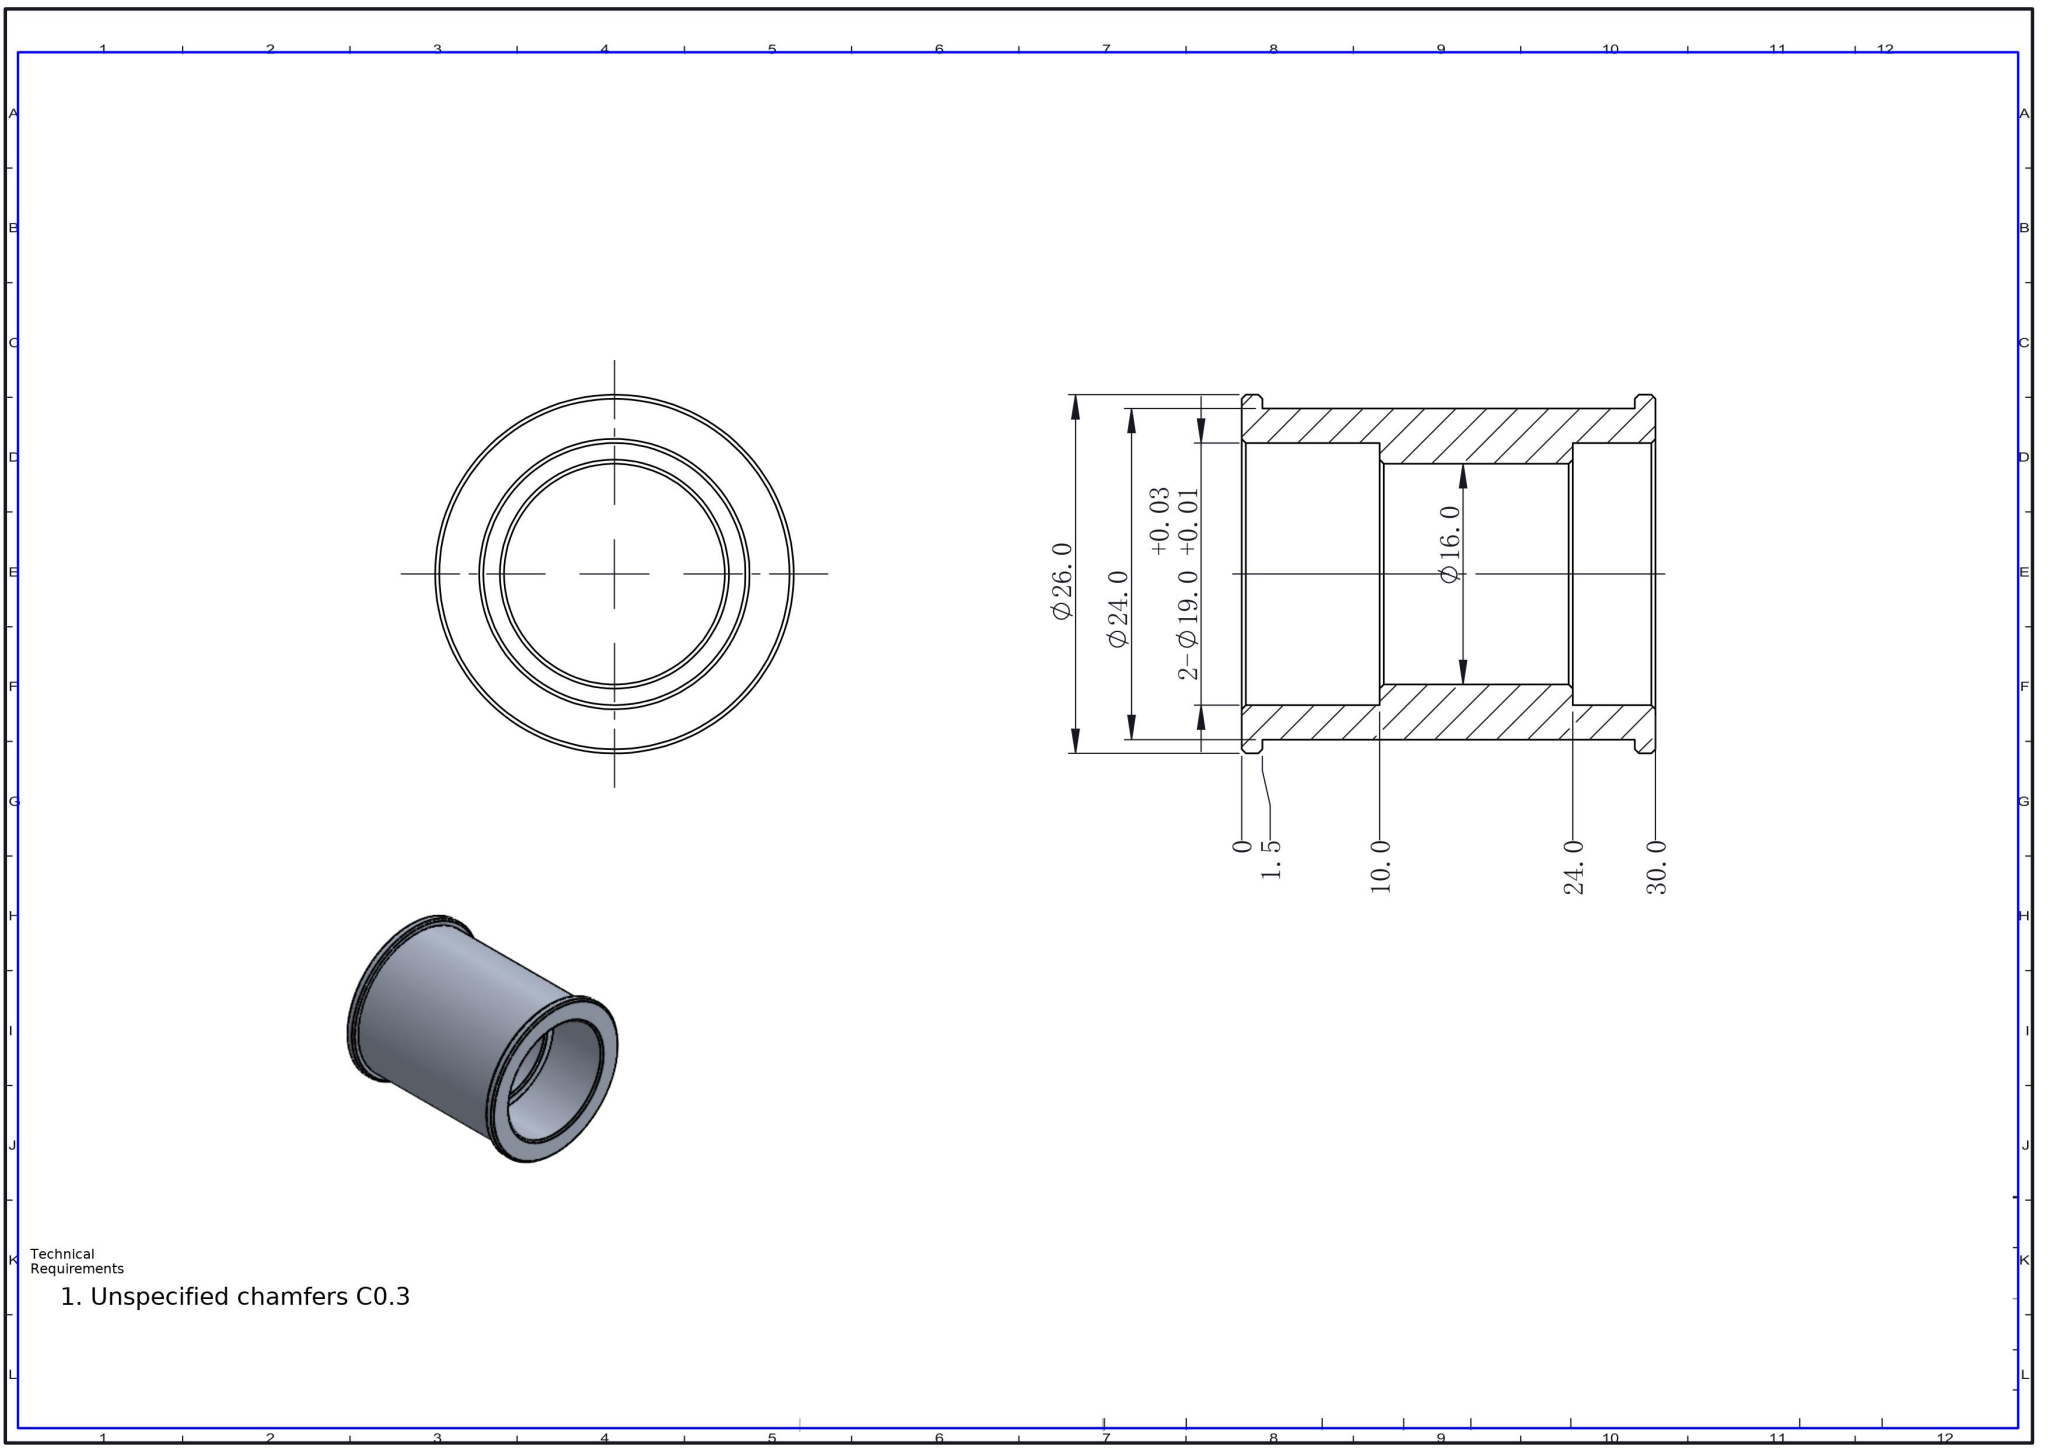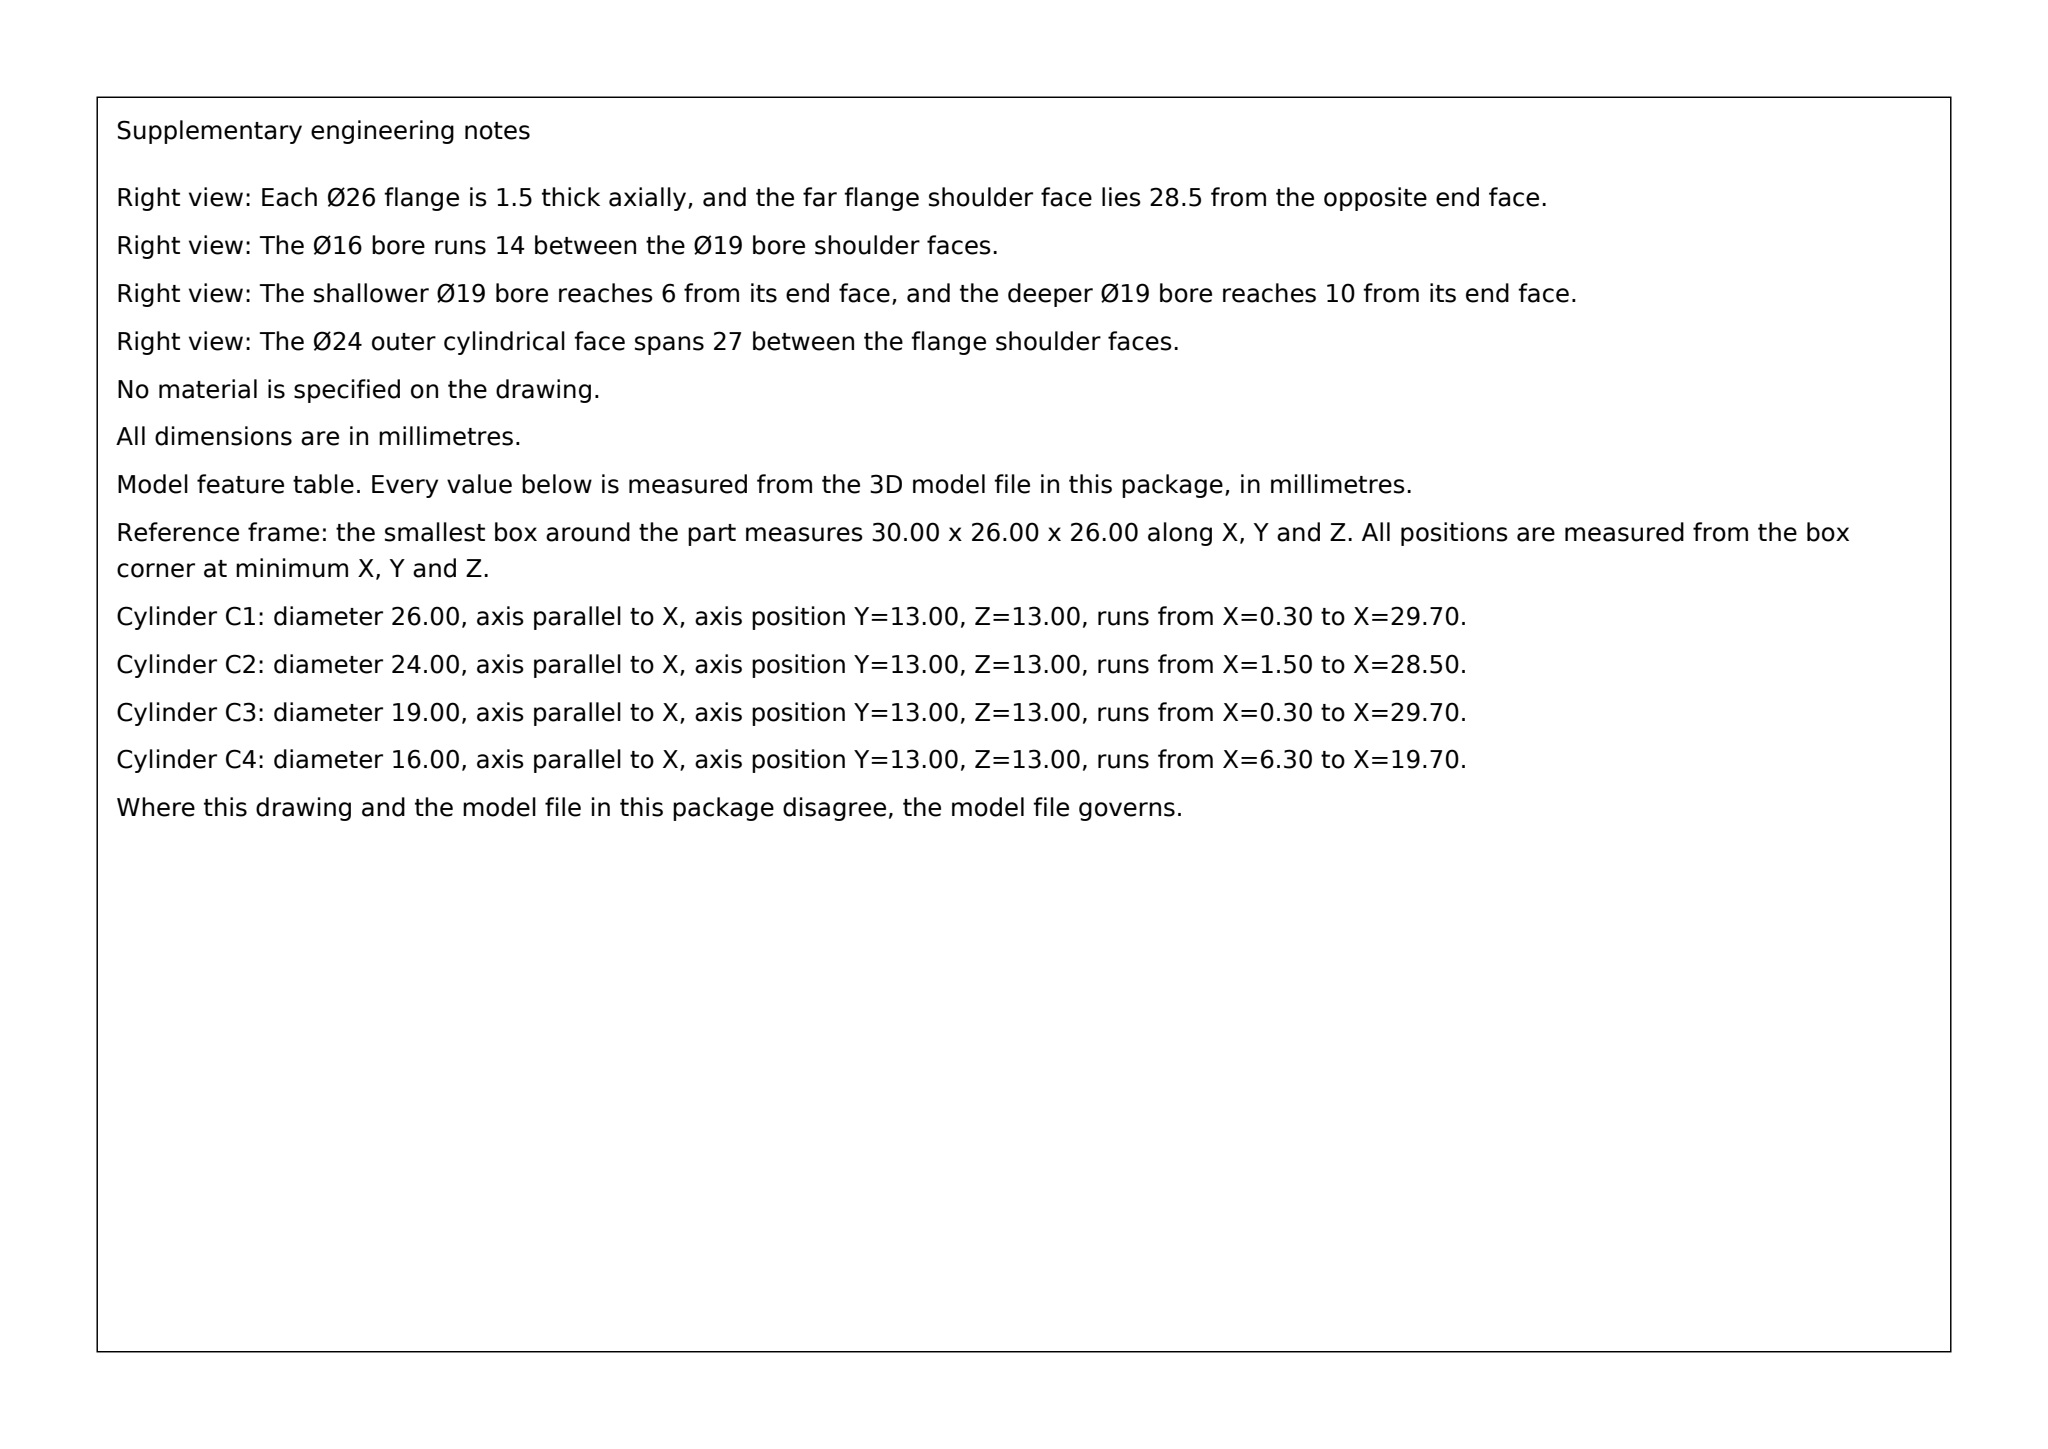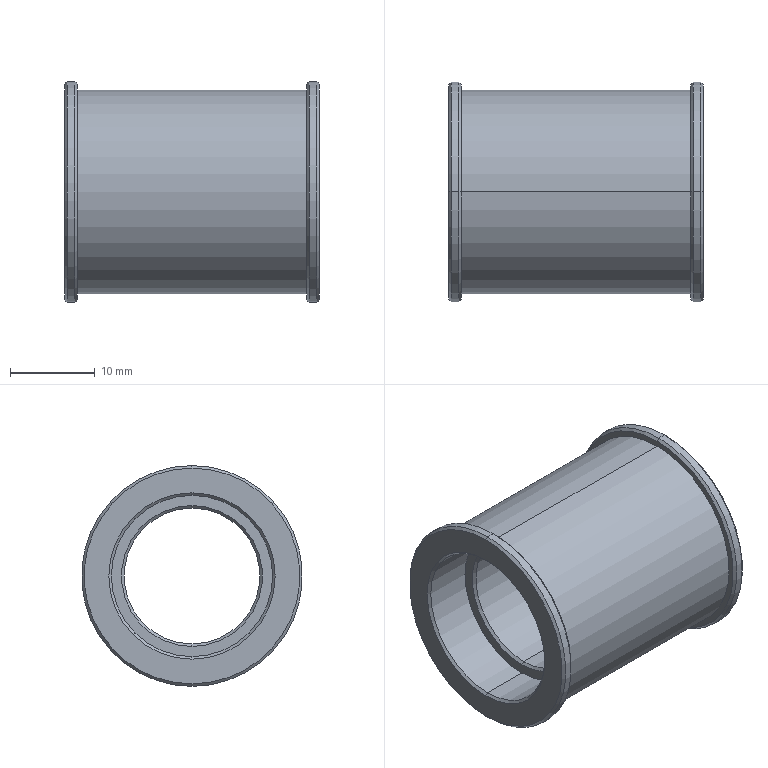Part | SolidWorks | mm | 1 solid | 34 faces | box 30 x 26 x 26 mm | volume 6431 mm3 | cone 16 | cylinder 12 | plane 6 | commonest cylinder face diameters 19 x4 26 x4 24 x2 16 x2
Drawing notes:
Ø26 COLLAR 1.5 WIDE EA END (0-1.5 & 28.5-30), C0.3 CHAM | from the solid: Ø26 cyl on x-axis at both ends; planes x=0/1.5 and x=28.5/30; 90 deg cones ref dia 26 & 25.4 (4 ea) give C0.3 breaks; Ø24 body 27 long between
build123d program:
from build123d import *

# Parameters (mm, degrees)
CHAMFER1_SIZE = 0.3


with BuildPart() as part:
    # Sketch1 → Revolve1 (revolve)
    with BuildSketch(Plane.XY, mode=Mode.PRIVATE) as revolve1_sk:
        Polygon((7, 8), (-7, 8), (-7, 9.5), (-13, 9.5), (-13, 13), (-11.5, 13), (-11.5, 12), (15.5, 12), (15.5, 13), (17, 13), (17, 9.5), (7, 9.5), align=None)
    revolve(revolve1_sk.sketch.rotate(Axis((0, 0, 0), (1, 0, 0)), 90), axis=Axis((0, 0, 0), (1, 0, 0)))

    # Chamfer1
    chamfer1_edges = [part.edges().sort_by_distance(p)[0] for p in [
        (17, 0, -13),
        (15.5, 0, -13),
        (-11.5, 0, -13),
        (-13, 0, -13),
        (-13, 0, -9.5),
        (-7, 0, -8),
        (7, 0, -8),
        (17, 0, -9.5),
    ]]
    chamfer(chamfer1_edges, length=CHAMFER1_SIZE)


solid = part.part
STEP:
#1=CARTESIAN_POINT('',(-13.,0.,12.7));
#2=VERTEX_POINT('',#1);
#3=CARTESIAN_POINT('',(-13.,0.,-12.7));
#4=VERTEX_POINT('',#3);
#5=CARTESIAN_POINT('',(-13.,0.,0.));
#6=DIRECTION('',(-1.,0.,0.));
#7=DIRECTION('',(0.,0.,-1.));
#8=AXIS2_PLACEMENT_3D('',#5,#6,#7);
#9=CIRCLE('',#8,12.7);
#10=EDGE_CURVE('',#2,#4,#9,.T.);
#11=ORIENTED_EDGE('',*,*,#10,.F.);
#12=CARTESIAN_POINT('',(-12.7,0.,13.));
#13=VERTEX_POINT('',#12);
#14=CARTESIAN_POINT('',(-13.,0.,12.7));
#15=DIRECTION('',(0.7071,0.,0.7071));
#16=VECTOR('',#15,1000.);
#17=LINE('',#14,#16);
#18=EDGE_CURVE('',#2,#13,#17,.T.);
#19=ORIENTED_EDGE('',*,*,#18,.T.);
#20=CARTESIAN_POINT('',(-12.7,0.,-13.));
#21=VERTEX_POINT('',#20);
#22=CARTESIAN_POINT('',(-12.7,0.,0.));
#23=DIRECTION('',(1.,0.,0.));
#24=DIRECTION('',(0.,0.,-1.));
#25=AXIS2_PLACEMENT_3D('',#22,#23,#24);
#26=CIRCLE('',#25,13.);
#27=EDGE_CURVE('',#21,#13,#26,.T.);
#28=ORIENTED_EDGE('',*,*,#27,.F.);
#29=CARTESIAN_POINT('',(-13.,0.,-12.7));
#30=DIRECTION('',(0.7071,0.,-0.7071));
#31=VECTOR('',#30,1000.);
#32=LINE('',#29,#31);
#33=EDGE_CURVE('',#4,#21,#32,.T.);
#34=ORIENTED_EDGE('',*,*,#33,.F.);
#35=EDGE_LOOP('',(#11,#19,#28,#34));
#36=FACE_OUTER_BOUND('',#35,.T.);
#37=CARTESIAN_POINT('',(-13.,0.,0.));
#38=DIRECTION('',(1.,0.,0.));
#39=DIRECTION('',(0.,0.,-1.));
#40=AXIS2_PLACEMENT_3D('',#37,#38,#39);
#41=CONICAL_SURFACE('',#40,12.7,0.7854);
#42=ADVANCED_FACE('',(#36),#41,.T.);
#43=CARTESIAN_POINT('',(-12.7,0.,-9.5));
#44=VERTEX_POINT('',#43);
#45=CARTESIAN_POINT('',(-12.7,0.,9.5));
#46=VERTEX_POINT('',#45);
#47=CARTESIAN_POINT('',(-12.7,0.,0.));
#48=DIRECTION('',(-1.,0.,0.));
#49=DIRECTION('',(0.,0.,-1.));
#50=AXIS2_PLACEMENT_3D('',#47,#48,#49);
#51=CIRCLE('',#50,9.5);
#52=EDGE_CURVE('',#44,#46,#51,.T.);
#53=ORIENTED_EDGE('',*,*,#52,.F.);
#54=CARTESIAN_POINT('',(-13.,0.,-9.8));
#55=VERTEX_POINT('',#54);
#56=CARTESIAN_POINT('',(-12.7,0.,-9.5));
#57=DIRECTION('',(-0.7071,0.,-0.7071));
#58=VECTOR('',#57,1000.);
#59=LINE('',#56,#58);
#60=EDGE_CURVE('',#44,#55,#59,.T.);
#61=ORIENTED_EDGE('',*,*,#60,.T.);
#62=CARTESIAN_POINT('',(-13.,0.,9.8));
#63=VERTEX_POINT('',#62);
#64=CARTESIAN_POINT('',(-13.,0.,0.));
#65=DIRECTION('',(1.,0.,0.));
#66=DIRECTION('',(0.,0.,-1.));
#67=AXIS2_PLACEMENT_3D('',#64,#65,#66);
#68=CIRCLE('',#67,9.8);
#69=EDGE_CURVE('',#63,#55,#68,.T.);
#70=ORIENTED_EDGE('',*,*,#69,.F.);
#71=CARTESIAN_POINT('',(-12.7,0.,9.5));
#72=DIRECTION('',(-0.7071,0.,0.7071));
#73=VECTOR('',#72,1000.);
#74=LINE('',#71,#73);
#75=EDGE_CURVE('',#46,#63,#74,.T.);
#76=ORIENTED_EDGE('',*,*,#75,.F.);
#77=EDGE_LOOP('',(#53,#61,#70,#76));
#78=FACE_OUTER_BOUND('',#77,.T.);
#79=CARTESIAN_POINT('',(-12.7,0.,0.));
#80=DIRECTION('',(-1.,0.,0.));
#81=DIRECTION('',(0.,0.,1.));
#82=AXIS2_PLACEMENT_3D('',#79,#80,#81);
#83=CONICAL_SURFACE('',#82,9.5,0.7854);
#84=ADVANCED_FACE('',(#78),#83,.F.);
#85=CARTESIAN_POINT('',(-6.7,0.,-8.));
#86=VERTEX_POINT('',#85);
#87=CARTESIAN_POINT('',(-6.7,0.,8.));
#88=VERTEX_POINT('',#87);
#89=CARTESIAN_POINT('',(-6.7,0.,0.));
#90=DIRECTION('',(-1.,0.,0.));
#91=DIRECTION('',(0.,0.,-1.));
#92=AXIS2_PLACEMENT_3D('',#89,#90,#91);
#93=CIRCLE('',#92,8.);
#94=EDGE_CURVE('',#86,#88,#93,.T.);
#95=ORIENTED_EDGE('',*,*,#94,.F.);
#96=CARTESIAN_POINT('',(-7.,0.,-8.3));
#97=VERTEX_POINT('',#96);
#98=CARTESIAN_POINT('',(-6.7,0.,-8.));
#99=DIRECTION('',(-0.7071,0.,-0.7071));
#100=VECTOR('',#99,1000.);
#101=LINE('',#98,#100);
#102=EDGE_CURVE('',#86,#97,#101,.T.);
#103=ORIENTED_EDGE('',*,*,#102,.T.);
#104=CARTESIAN_POINT('',(-7.,0.,8.3));
#105=VERTEX_POINT('',#104);
#106=CARTESIAN_POINT('',(-7.,0.,0.));
#107=DIRECTION('',(1.,0.,0.));
#108=DIRECTION('',(0.,0.,-1.));
#109=AXIS2_PLACEMENT_3D('',#106,#107,#108);
#110=CIRCLE('',#109,8.3);
#111=EDGE_CURVE('',#105,#97,#110,.T.);
#112=ORIENTED_EDGE('',*,*,#111,.F.);
#113=CARTESIAN_POINT('',(-6.7,0.,8.));
#114=DIRECTION('',(-0.7071,0.,0.7071));
#115=VECTOR('',#114,1000.);
#116=LINE('',#113,#115);
#117=EDGE_CURVE('',#88,#105,#116,.T.);
#118=ORIENTED_EDGE('',*,*,#117,.F.);
#119=EDGE_LOOP('',(#95,#103,#112,#118));
#120=FACE_OUTER_BOUND('',#119,.T.);
#121=CARTESIAN_POINT('',(-6.7,0.,0.));
#122=DIRECTION('',(-1.,0.,0.));
#123=DIRECTION('',(0.,0.,1.));
#124=AXIS2_PLACEMENT_3D('',#121,#122,#123);
#125=CONICAL_SURFACE('',#124,8.,0.7854);
#126=ADVANCED_FACE('',(#120),#125,.F.);
#127=CARTESIAN_POINT('',(16.7,0.,9.5));
#128=VERTEX_POINT('',#127);
#129=CARTESIAN_POINT('',(16.7,0.,-9.5));
#130=VERTEX_POINT('',#129);
#131=CARTESIAN_POINT('',(16.7,0.,0.));
#132=DIRECTION('',(1.,0.,0.));
#133=DIRECTION('',(0.,0.,1.));
#134=AXIS2_PLACEMENT_3D('',#131,#132,#133);
#135=CIRCLE('',#134,9.5);
#136=EDGE_CURVE('',#128,#130,#135,.T.);
#137=ORIENTED_EDGE('',*,*,#136,.F.);
#138=CARTESIAN_POINT('',(17.,0.,9.8));
#139=VERTEX_POINT('',#138);
#140=CARTESIAN_POINT('',(17.,0.,9.8));
#141=DIRECTION('',(0.7071,0.,0.7071));
#142=VECTOR('',#141,1000.);
#143=LINE('',#140,#142);
#144=EDGE_CURVE('',#128,#139,#143,.T.);
#145=ORIENTED_EDGE('',*,*,#144,.T.);
#146=CARTESIAN_POINT('',(17.,0.,-9.8));
#147=VERTEX_POINT('',#146);
#148=CARTESIAN_POINT('',(17.,0.,0.));
#149=DIRECTION('',(-1.,0.,0.));
#150=DIRECTION('',(0.,0.,1.));
#151=AXIS2_PLACEMENT_3D('',#148,#149,#150);
#152=CIRCLE('',#151,9.8);
#153=EDGE_CURVE('',#147,#139,#152,.T.);
#154=ORIENTED_EDGE('',*,*,#153,.F.);
#155=CARTESIAN_POINT('',(17.,0.,-9.8));
#156=DIRECTION('',(0.7071,0.,-0.7071));
#157=VECTOR('',#156,1000.);
#158=LINE('',#155,#157);
#159=EDGE_CURVE('',#130,#147,#158,.T.);
#160=ORIENTED_EDGE('',*,*,#159,.F.);
#161=EDGE_LOOP('',(#137,#145,#154,#160));
#162=FACE_OUTER_BOUND('',#161,.T.);
#163=CARTESIAN_POINT('',(17.,0.,0.));
#164=DIRECTION('',(1.,0.,0.));
#165=DIRECTION('',(0.,0.,-1.));
#166=AXIS2_PLACEMENT_3D('',#163,#164,#165);
#167=CONICAL_SURFACE('',#166,9.8,0.7854);
#168=ADVANCED_FACE('',(#162),#167,.F.);
#169=CARTESIAN_POINT('',(17.,0.,-12.7));
#170=VERTEX_POINT('',#169);
#171=CARTESIAN_POINT('',(17.,0.,12.7));
#172=VERTEX_POINT('',#171);
#173=CARTESIAN_POINT('',(17.,0.,0.));
#174=DIRECTION('',(1.,0.,0.));
#175=DIRECTION('',(0.,0.,1.));
#176=AXIS2_PLACEMENT_3D('',#173,#174,#175);
#177=CIRCLE('',#176,12.7);
#178=EDGE_CURVE('',#170,#172,#177,.T.);
#179=ORIENTED_EDGE('',*,*,#178,.F.);
#180=CARTESIAN_POINT('',(16.7,0.,-13.));
#181=VERTEX_POINT('',#180);
#182=CARTESIAN_POINT('',(16.7,0.,-13.));
#183=DIRECTION('',(-0.7071,0.,-0.7071));
#184=VECTOR('',#183,1000.);
#185=LINE('',#182,#184);
#186=EDGE_CURVE('',#170,#181,#185,.T.);
#187=ORIENTED_EDGE('',*,*,#186,.T.);
#188=CARTESIAN_POINT('',(16.7,0.,13.));
#189=VERTEX_POINT('',#188);
#190=CARTESIAN_POINT('',(16.7,0.,0.));
#191=DIRECTION('',(-1.,0.,0.));
#192=DIRECTION('',(0.,0.,1.));
#193=AXIS2_PLACEMENT_3D('',#190,#191,#192);
#194=CIRCLE('',#193,13.);
#195=EDGE_CURVE('',#189,#181,#194,.T.);
#196=ORIENTED_EDGE('',*,*,#195,.F.);
#197=CARTESIAN_POINT('',(16.7,0.,13.));
#198=DIRECTION('',(-0.7071,0.,0.7071));
#199=VECTOR('',#198,1000.);
#200=LINE('',#197,#199);
#201=EDGE_CURVE('',#172,#189,#200,.T.);
#202=ORIENTED_EDGE('',*,*,#201,.F.);
#203=EDGE_LOOP('',(#179,#187,#196,#202));
#204=FACE_OUTER_BOUND('',#203,.T.);
#205=CARTESIAN_POINT('',(16.7,0.,0.));
#206=DIRECTION('',(-1.,0.,0.));
#207=DIRECTION('',(0.,0.,1.));
#208=AXIS2_PLACEMENT_3D('',#205,#206,#207);
#209=CONICAL_SURFACE('',#208,13.,0.7854);
#210=ADVANCED_FACE('',(#204),#209,.T.);
#211=CARTESIAN_POINT('',(15.5,0.,12.7));
#212=VERTEX_POINT('',#211);
#213=CARTESIAN_POINT('',(15.5,0.,-12.7));
#214=VERTEX_POINT('',#213);
#215=CARTESIAN_POINT('',(15.5,0.,0.));
#216=DIRECTION('',(-1.,0.,0.));
#217=DIRECTION('',(0.,0.,-1.));
#218=AXIS2_PLACEMENT_3D('',#215,#216,#217);
#219=CIRCLE('',#218,12.7);
#220=EDGE_CURVE('',#212,#214,#219,.T.);
#221=ORIENTED_EDGE('',*,*,#220,.F.);
#222=CARTESIAN_POINT('',(15.8,0.,13.));
#223=VERTEX_POINT('',#222);
#224=CARTESIAN_POINT('',(15.5,0.,12.7));
#225=DIRECTION('',(0.7071,0.,0.7071));
#226=VECTOR('',#225,1000.);
#227=LINE('',#224,#226);
#228=EDGE_CURVE('',#212,#223,#227,.T.);
#229=ORIENTED_EDGE('',*,*,#228,.T.);
#230=CARTESIAN_POINT('',(15.8,0.,-13.));
#231=VERTEX_POINT('',#230);
#232=CARTESIAN_POINT('',(15.8,0.,0.));
#233=DIRECTION('',(1.,0.,0.));
#234=DIRECTION('',(0.,0.,-1.));
#235=AXIS2_PLACEMENT_3D('',#232,#233,#234);
#236=CIRCLE('',#235,13.);
#237=EDGE_CURVE('',#231,#223,#236,.T.);
#238=ORIENTED_EDGE('',*,*,#237,.F.);
#239=CARTESIAN_POINT('',(15.5,0.,-12.7));
#240=DIRECTION('',(0.7071,0.,-0.7071));
#241=VECTOR('',#240,1000.);
#242=LINE('',#239,#241);
#243=EDGE_CURVE('',#214,#231,#242,.T.);
#244=ORIENTED_EDGE('',*,*,#243,.F.);
#245=EDGE_LOOP('',(#221,#229,#238,#244));
#246=FACE_OUTER_BOUND('',#245,.T.);
#247=CARTESIAN_POINT('',(15.5,0.,0.));
#248=DIRECTION('',(1.,0.,0.));
#249=DIRECTION('',(0.,0.,-1.));
#250=AXIS2_PLACEMENT_3D('',#247,#248,#249);
#251=CONICAL_SURFACE('',#250,12.7,0.7854);
#252=ADVANCED_FACE('',(#246),#251,.T.);
#253=CARTESIAN_POINT('',(6.7,0.,8.));
#254=VERTEX_POINT('',#253);
#255=CARTESIAN_POINT('',(6.7,0.,-8.));
#256=VERTEX_POINT('',#255);
#257=CARTESIAN_POINT('',(6.7,0.,0.));
#258=DIRECTION('',(1.,0.,0.));
#259=DIRECTION('',(0.,0.,1.));
#260=AXIS2_PLACEMENT_3D('',#257,#258,#259);
#261=CIRCLE('',#260,8.);
#262=EDGE_CURVE('',#254,#256,#261,.T.);
#263=ORIENTED_EDGE('',*,*,#262,.F.);
#264=CARTESIAN_POINT('',(7.,0.,8.3));
#265=VERTEX_POINT('',#264);
#266=CARTESIAN_POINT('',(7.,0.,8.3));
#267=DIRECTION('',(0.7071,0.,0.7071));
#268=VECTOR('',#267,1000.);
#269=LINE('',#266,#268);
#270=EDGE_CURVE('',#254,#265,#269,.T.);
#271=ORIENTED_EDGE('',*,*,#270,.T.);
#272=CARTESIAN_POINT('',(7.,0.,-8.3));
#273=VERTEX_POINT('',#272);
#274=CARTESIAN_POINT('',(7.,0.,0.));
#275=DIRECTION('',(-1.,0.,0.));
#276=DIRECTION('',(0.,0.,1.));
#277=AXIS2_PLACEMENT_3D('',#274,#275,#276);
#278=CIRCLE('',#277,8.3);
#279=EDGE_CURVE('',#273,#265,#278,.T.);
#280=ORIENTED_EDGE('',*,*,#279,.F.);
#281=CARTESIAN_POINT('',(7.,0.,-8.3));
#282=DIRECTION('',(0.7071,0.,-0.7071));
#283=VECTOR('',#282,1000.);
#284=LINE('',#281,#283);
#285=EDGE_CURVE('',#256,#273,#284,.T.);
#286=ORIENTED_EDGE('',*,*,#285,.F.);
#287=EDGE_LOOP('',(#263,#271,#280,#286));
#288=FACE_OUTER_BOUND('',#287,.T.);
#289=CARTESIAN_POINT('',(7.,0.,0.));
#290=DIRECTION('',(1.,0.,0.));
#291=DIRECTION('',(0.,0.,-1.));
#292=AXIS2_PLACEMENT_3D('',#289,#290,#291);
#293=CONICAL_SURFACE('',#292,8.3,0.7854);
#294=ADVANCED_FACE('',(#288),#293,.F.);
#295=CARTESIAN_POINT('',(-11.5,0.,-12.7));
#296=VERTEX_POINT('',#295);
#297=CARTESIAN_POINT('',(-11.5,0.,12.7));
#298=VERTEX_POINT('',#297);
#299=CARTESIAN_POINT('',(-11.5,0.,0.));
#300=DIRECTION('',(1.,0.,0.));
#301=DIRECTION('',(0.,0.,1.));
#302=AXIS2_PLACEMENT_3D('',#299,#300,#301);
#303=CIRCLE('',#302,12.7);
#304=EDGE_CURVE('',#296,#298,#303,.T.);
#305=ORIENTED_EDGE('',*,*,#304,.F.);
#306=CARTESIAN_POINT('',(-11.8,0.,-13.));
#307=VERTEX_POINT('',#306);
#308=CARTESIAN_POINT('',(-11.8,0.,-13.));
#309=DIRECTION('',(-0.7071,0.,-0.7071));
#310=VECTOR('',#309,1000.);
#311=LINE('',#308,#310);
#312=EDGE_CURVE('',#296,#307,#311,.T.);
#313=ORIENTED_EDGE('',*,*,#312,.T.);
#314=CARTESIAN_POINT('',(-11.8,0.,13.));
#315=VERTEX_POINT('',#314);
#316=CARTESIAN_POINT('',(-11.8,0.,0.));
#317=DIRECTION('',(-1.,0.,0.));
#318=DIRECTION('',(0.,0.,1.));
#319=AXIS2_PLACEMENT_3D('',#316,#317,#318);
#320=CIRCLE('',#319,13.);
#321=EDGE_CURVE('',#315,#307,#320,.T.);
#322=ORIENTED_EDGE('',*,*,#321,.F.);
#323=CARTESIAN_POINT('',(-11.8,0.,13.));
#324=DIRECTION('',(-0.7071,0.,0.7071));
#325=VECTOR('',#324,1000.);
#326=LINE('',#323,#325);
#327=EDGE_CURVE('',#298,#315,#326,.T.);
#328=ORIENTED_EDGE('',*,*,#327,.F.);
#329=EDGE_LOOP('',(#305,#313,#322,#328));
#330=FACE_OUTER_BOUND('',#329,.T.);
#331=CARTESIAN_POINT('',(-11.8,0.,0.));
#332=DIRECTION('',(-1.,0.,0.));
#333=DIRECTION('',(0.,0.,1.));
#334=AXIS2_PLACEMENT_3D('',#331,#332,#333);
#335=CONICAL_SURFACE('',#334,13.,0.7854);
#336=ADVANCED_FACE('',(#330),#335,.T.);
#337=ORIENTED_EDGE('',*,*,#136,.T.);
#338=CARTESIAN_POINT('',(7.,0.,-9.5));
#339=VERTEX_POINT('',#338);
#340=CARTESIAN_POINT('',(0.,0.,-9.5));
#341=DIRECTION('',(-1.,0.,0.));
#342=VECTOR('',#341,1000.);
#343=LINE('',#340,#342);
#344=EDGE_CURVE('',#130,#339,#343,.T.);
#345=ORIENTED_EDGE('',*,*,#344,.T.);
#346=CARTESIAN_POINT('',(7.,0.,9.5));
#347=VERTEX_POINT('',#346);
#348=CARTESIAN_POINT('',(7.,0.,0.));
#349=DIRECTION('',(-1.,0.,0.));
#350=DIRECTION('',(0.,0.,1.));
#351=AXIS2_PLACEMENT_3D('',#348,#349,#350);
#352=CIRCLE('',#351,9.5);
#353=EDGE_CURVE('',#339,#347,#352,.T.);
#354=ORIENTED_EDGE('',*,*,#353,.T.);
#355=CARTESIAN_POINT('',(0.,0.,9.5));
#356=DIRECTION('',(-1.,0.,0.));
#357=VECTOR('',#356,1000.);
#358=LINE('',#355,#357);
#359=EDGE_CURVE('',#128,#347,#358,.T.);
#360=ORIENTED_EDGE('',*,*,#359,.F.);
#361=EDGE_LOOP('',(#337,#345,#354,#360));
#362=FACE_OUTER_BOUND('',#361,.T.);
#363=CARTESIAN_POINT('',(0.,0.,0.));
#364=DIRECTION('',(-1.,0.,0.));
#365=DIRECTION('',(0.,0.,1.));
#366=AXIS2_PLACEMENT_3D('',#363,#364,#365);
#367=CYLINDRICAL_SURFACE('',#366,9.5);
#368=ADVANCED_FACE('',(#362),#367,.F.);
#369=ORIENTED_EDGE('',*,*,#195,.T.);
#370=CARTESIAN_POINT('',(0.,0.,-13.));
#371=DIRECTION('',(-1.,0.,0.));
#372=VECTOR('',#371,1000.);
#373=LINE('',#370,#372);
#374=EDGE_CURVE('',#181,#231,#373,.T.);
#375=ORIENTED_EDGE('',*,*,#374,.T.);
#376=ORIENTED_EDGE('',*,*,#237,.T.);
#377=CARTESIAN_POINT('',(0.,0.,13.));
#378=DIRECTION('',(-1.,0.,0.));
#379=VECTOR('',#378,1000.);
#380=LINE('',#377,#379);
#381=EDGE_CURVE('',#189,#223,#380,.T.);
#382=ORIENTED_EDGE('',*,*,#381,.F.);
#383=EDGE_LOOP('',(#369,#375,#376,#382));
#384=FACE_OUTER_BOUND('',#383,.T.);
#385=CARTESIAN_POINT('',(0.,0.,0.));
#386=DIRECTION('',(-1.,0.,0.));
#387=DIRECTION('',(0.,0.,1.));
#388=AXIS2_PLACEMENT_3D('',#385,#386,#387);
#389=CYLINDRICAL_SURFACE('',#388,13.);
#390=ADVANCED_FACE('',(#384),#389,.T.);
#391=CARTESIAN_POINT('',(15.5,0.,12.));
#392=VERTEX_POINT('',#391);
#393=CARTESIAN_POINT('',(15.5,0.,-12.));
#394=VERTEX_POINT('',#393);
#395=CARTESIAN_POINT('',(15.5,0.,0.));
#396=DIRECTION('',(-1.,0.,0.));
#397=DIRECTION('',(0.,0.,1.));
#398=AXIS2_PLACEMENT_3D('',#395,#396,#397);
#399=CIRCLE('',#398,12.);
#400=EDGE_CURVE('',#392,#394,#399,.T.);
#401=ORIENTED_EDGE('',*,*,#400,.T.);
#402=CARTESIAN_POINT('',(-11.5,0.,-12.));
#403=VERTEX_POINT('',#402);
#404=CARTESIAN_POINT('',(0.,0.,-12.));
#405=DIRECTION('',(-1.,0.,0.));
#406=VECTOR('',#405,1000.);
#407=LINE('',#404,#406);
#408=EDGE_CURVE('',#394,#403,#407,.T.);
#409=ORIENTED_EDGE('',*,*,#408,.T.);
#410=CARTESIAN_POINT('',(-11.5,0.,12.));
#411=VERTEX_POINT('',#410);
#412=CARTESIAN_POINT('',(-11.5,0.,0.));
#413=DIRECTION('',(-1.,0.,0.));
#414=DIRECTION('',(0.,0.,1.));
#415=AXIS2_PLACEMENT_3D('',#412,#413,#414);
#416=CIRCLE('',#415,12.);
#417=EDGE_CURVE('',#411,#403,#416,.T.);
#418=ORIENTED_EDGE('',*,*,#417,.F.);
#419=CARTESIAN_POINT('',(0.,0.,12.));
#420=DIRECTION('',(-1.,0.,0.));
#421=VECTOR('',#420,1000.);
#422=LINE('',#419,#421);
#423=EDGE_CURVE('',#392,#411,#422,.T.);
#424=ORIENTED_EDGE('',*,*,#423,.F.);
#425=EDGE_LOOP('',(#401,#409,#418,#424));
#426=FACE_OUTER_BOUND('',#425,.T.);
#427=CARTESIAN_POINT('',(0.,0.,0.));
#428=DIRECTION('',(-1.,0.,0.));
#429=DIRECTION('',(0.,0.,1.));
#430=AXIS2_PLACEMENT_3D('',#427,#428,#429);
#431=CYLINDRICAL_SURFACE('',#430,12.);
#432=ADVANCED_FACE('',(#426),#431,.T.);
#433=ORIENTED_EDGE('',*,*,#321,.T.);
#434=CARTESIAN_POINT('',(0.,0.,-13.));
#435=DIRECTION('',(-1.,0.,0.));
#436=VECTOR('',#435,1000.);
#437=LINE('',#434,#436);
#438=EDGE_CURVE('',#307,#21,#437,.T.);
#439=ORIENTED_EDGE('',*,*,#438,.T.);
#440=ORIENTED_EDGE('',*,*,#27,.T.);
#441=CARTESIAN_POINT('',(0.,0.,13.));
#442=DIRECTION('',(-1.,0.,0.));
#443=VECTOR('',#442,1000.);
#444=LINE('',#441,#443);
#445=EDGE_CURVE('',#315,#13,#444,.T.);
#446=ORIENTED_EDGE('',*,*,#445,.F.);
#447=EDGE_LOOP('',(#433,#439,#440,#446));
#448=FACE_OUTER_BOUND('',#447,.T.);
#449=CARTESIAN_POINT('',(0.,0.,0.));
#450=DIRECTION('',(-1.,0.,0.));
#451=DIRECTION('',(0.,0.,1.));
#452=AXIS2_PLACEMENT_3D('',#449,#450,#451);
#453=CYLINDRICAL_SURFACE('',#452,13.);
#454=ADVANCED_FACE('',(#448),#453,.T.);
#455=CARTESIAN_POINT('',(-7.,0.,-9.5));
#456=VERTEX_POINT('',#455);
#457=CARTESIAN_POINT('',(-7.,0.,9.5));
#458=VERTEX_POINT('',#457);
#459=CARTESIAN_POINT('',(-7.,0.,0.));
#460=DIRECTION('',(-1.,0.,0.));
#461=DIRECTION('',(0.,0.,1.));
#462=AXIS2_PLACEMENT_3D('',#459,#460,#461);
#463=CIRCLE('',#462,9.5);
#464=EDGE_CURVE('',#456,#458,#463,.T.);
#465=ORIENTED_EDGE('',*,*,#464,.F.);
#466=CARTESIAN_POINT('',(0.,0.,-9.5));
#467=DIRECTION('',(-1.,0.,0.));
#468=VECTOR('',#467,1000.);
#469=LINE('',#466,#468);
#470=EDGE_CURVE('',#456,#44,#469,.T.);
#471=ORIENTED_EDGE('',*,*,#470,.T.);
#472=ORIENTED_EDGE('',*,*,#52,.T.);
#473=CARTESIAN_POINT('',(0.,0.,9.5));
#474=DIRECTION('',(-1.,0.,0.));
#475=VECTOR('',#474,1000.);
#476=LINE('',#473,#475);
#477=EDGE_CURVE('',#458,#46,#476,.T.);
#478=ORIENTED_EDGE('',*,*,#477,.F.);
#479=EDGE_LOOP('',(#465,#471,#472,#478));
#480=FACE_OUTER_BOUND('',#479,.T.);
#481=CARTESIAN_POINT('',(0.,0.,0.));
#482=DIRECTION('',(-1.,0.,0.));
#483=DIRECTION('',(0.,0.,1.));
#484=AXIS2_PLACEMENT_3D('',#481,#482,#483);
#485=CYLINDRICAL_SURFACE('',#484,9.5);
#486=ADVANCED_FACE('',(#480),#485,.F.);
#487=ORIENTED_EDGE('',*,*,#262,.T.);
#488=CARTESIAN_POINT('',(0.,0.,-8.));
#489=DIRECTION('',(-1.,0.,0.));
#490=VECTOR('',#489,1000.);
#491=LINE('',#488,#490);
#492=EDGE_CURVE('',#256,#86,#491,.T.);
#493=ORIENTED_EDGE('',*,*,#492,.T.);
#494=ORIENTED_EDGE('',*,*,#94,.T.);
#495=CARTESIAN_POINT('',(0.,0.,8.));
#496=DIRECTION('',(-1.,0.,0.));
#497=VECTOR('',#496,1000.);
#498=LINE('',#495,#497);
#499=EDGE_CURVE('',#254,#88,#498,.T.);
#500=ORIENTED_EDGE('',*,*,#499,.F.);
#501=EDGE_LOOP('',(#487,#493,#494,#500));
#502=FACE_OUTER_BOUND('',#501,.T.);
#503=CARTESIAN_POINT('',(0.,0.,0.));
#504=DIRECTION('',(-1.,0.,0.));
#505=DIRECTION('',(0.,0.,1.));
#506=AXIS2_PLACEMENT_3D('',#503,#504,#505);
#507=CYLINDRICAL_SURFACE('',#506,8.);
#508=ADVANCED_FACE('',(#502),#507,.F.);
#509=ORIENTED_EDGE('',*,*,#279,.T.);
#510=CARTESIAN_POINT('',(7.,0.,0.));
#511=DIRECTION('',(-1.,0.,0.));
#512=DIRECTION('',(0.,0.,1.));
#513=AXIS2_PLACEMENT_3D('',#510,#511,#512);
#514=CIRCLE('',#513,8.3);
#515=EDGE_CURVE('',#265,#273,#514,.T.);
#516=ORIENTED_EDGE('',*,*,#515,.T.);
#517=EDGE_LOOP('',(#509,#516));
#518=FACE_BOUND('',#517,.T.);
#519=CARTESIAN_POINT('',(7.,0.,0.));
#520=DIRECTION('',(-1.,0.,0.));
#521=DIRECTION('',(0.,0.,1.));
#522=AXIS2_PLACEMENT_3D('',#519,#520,#521);
#523=CIRCLE('',#522,9.5);
#524=EDGE_CURVE('',#347,#339,#523,.T.);
#525=ORIENTED_EDGE('',*,*,#524,.F.);
#526=ORIENTED_EDGE('',*,*,#353,.F.);
#527=EDGE_LOOP('',(#525,#526));
#528=FACE_OUTER_BOUND('',#527,.T.);
#529=CARTESIAN_POINT('',(7.,9.5,0.));
#530=DIRECTION('',(-1.,0.,0.));
#531=DIRECTION('',(0.,0.,1.));
#532=AXIS2_PLACEMENT_3D('',#529,#530,#531);
#533=PLANE('',#532);
#534=ADVANCED_FACE('',(#518,#528),#533,.F.);
#535=ORIENTED_EDGE('',*,*,#492,.F.);
#536=CARTESIAN_POINT('',(6.7,0.,0.));
#537=DIRECTION('',(1.,0.,0.));
#538=DIRECTION('',(0.,0.,1.));
#539=AXIS2_PLACEMENT_3D('',#536,#537,#538);
#540=CIRCLE('',#539,8.);
#541=EDGE_CURVE('',#256,#254,#540,.T.);
#542=ORIENTED_EDGE('',*,*,#541,.T.);
#543=ORIENTED_EDGE('',*,*,#499,.T.);
#544=CARTESIAN_POINT('',(-6.7,0.,0.));
#545=DIRECTION('',(-1.,0.,0.));
#546=DIRECTION('',(0.,0.,-1.));
#547=AXIS2_PLACEMENT_3D('',#544,#545,#546);
#548=CIRCLE('',#547,8.);
#549=EDGE_CURVE('',#88,#86,#548,.T.);
#550=ORIENTED_EDGE('',*,*,#549,.T.);
#551=EDGE_LOOP('',(#535,#542,#543,#550));
#552=FACE_OUTER_BOUND('',#551,.T.);
#553=CARTESIAN_POINT('',(0.,0.,0.));
#554=DIRECTION('',(-1.,0.,0.));
#555=DIRECTION('',(0.,0.,1.));
#556=AXIS2_PLACEMENT_3D('',#553,#554,#555);
#557=CYLINDRICAL_SURFACE('',#556,8.);
#558=ADVANCED_FACE('',(#552),#557,.F.);
#559=ORIENTED_EDGE('',*,*,#111,.T.);
#560=CARTESIAN_POINT('',(-7.,0.,0.));
#561=DIRECTION('',(1.,0.,0.));
#562=DIRECTION('',(0.,0.,-1.));
#563=AXIS2_PLACEMENT_3D('',#560,#561,#562);
#564=CIRCLE('',#563,8.3);
#565=EDGE_CURVE('',#97,#105,#564,.T.);
#566=ORIENTED_EDGE('',*,*,#565,.T.);
#567=EDGE_LOOP('',(#559,#566));
#568=FACE_BOUND('',#567,.T.);
#569=CARTESIAN_POINT('',(-7.,0.,0.));
#570=DIRECTION('',(-1.,0.,0.));
#571=DIRECTION('',(0.,0.,1.));
#572=AXIS2_PLACEMENT_3D('',#569,#570,#571);
#573=CIRCLE('',#572,9.5);
#574=EDGE_CURVE('',#458,#456,#573,.T.);
#575=ORIENTED_EDGE('',*,*,#574,.T.);
#576=ORIENTED_EDGE('',*,*,#464,.T.);
#577=EDGE_LOOP('',(#575,#576));
#578=FACE_OUTER_BOUND('',#577,.T.);
#579=CARTESIAN_POINT('',(-7.,8.,0.));
#580=DIRECTION('',(1.,0.,0.));
#581=DIRECTION('',(0.,0.,-1.));
#582=AXIS2_PLACEMENT_3D('',#579,#580,#581);
#583=PLANE('',#582);
#584=ADVANCED_FACE('',(#568,#578),#583,.F.);
#585=ORIENTED_EDGE('',*,*,#470,.F.);
#586=ORIENTED_EDGE('',*,*,#574,.F.);
#587=ORIENTED_EDGE('',*,*,#477,.T.);
#588=CARTESIAN_POINT('',(-12.7,0.,0.));
#589=DIRECTION('',(-1.,0.,0.));
#590=DIRECTION('',(0.,0.,-1.));
#591=AXIS2_PLACEMENT_3D('',#588,#589,#590);
#592=CIRCLE('',#591,9.5);
#593=EDGE_CURVE('',#46,#44,#592,.T.);
#594=ORIENTED_EDGE('',*,*,#593,.T.);
#595=EDGE_LOOP('',(#585,#586,#587,#594));
#596=FACE_OUTER_BOUND('',#595,.T.);
#597=CARTESIAN_POINT('',(0.,0.,0.));
#598=DIRECTION('',(-1.,0.,0.));
#599=DIRECTION('',(0.,0.,1.));
#600=AXIS2_PLACEMENT_3D('',#597,#598,#599);
#601=CYLINDRICAL_SURFACE('',#600,9.5);
#602=ADVANCED_FACE('',(#596),#601,.F.);
#603=ORIENTED_EDGE('',*,*,#69,.T.);
#604=CARTESIAN_POINT('',(-13.,0.,0.));
#605=DIRECTION('',(1.,0.,0.));
#606=DIRECTION('',(0.,0.,-1.));
#607=AXIS2_PLACEMENT_3D('',#604,#605,#606);
#608=CIRCLE('',#607,9.8);
#609=EDGE_CURVE('',#55,#63,#608,.T.);
#610=ORIENTED_EDGE('',*,*,#609,.T.);
#611=EDGE_LOOP('',(#603,#610));
#612=FACE_BOUND('',#611,.T.);
#613=CARTESIAN_POINT('',(-13.,0.,0.));
#614=DIRECTION('',(-1.,0.,0.));
#615=DIRECTION('',(0.,0.,-1.));
#616=AXIS2_PLACEMENT_3D('',#613,#614,#615);
#617=CIRCLE('',#616,12.7);
#618=EDGE_CURVE('',#4,#2,#617,.T.);
#619=ORIENTED_EDGE('',*,*,#618,.T.);
#620=ORIENTED_EDGE('',*,*,#10,.T.);
#621=EDGE_LOOP('',(#619,#620));
#622=FACE_OUTER_BOUND('',#621,.T.);
#623=CARTESIAN_POINT('',(-13.,9.5,0.));
#624=DIRECTION('',(1.,0.,0.));
#625=DIRECTION('',(0.,0.,-1.));
#626=AXIS2_PLACEMENT_3D('',#623,#624,#625);
#627=PLANE('',#626);
#628=ADVANCED_FACE('',(#612,#622),#627,.F.);
#629=ORIENTED_EDGE('',*,*,#438,.F.);
#630=CARTESIAN_POINT('',(-11.8,0.,0.));
#631=DIRECTION('',(-1.,0.,0.));
#632=DIRECTION('',(0.,0.,1.));
#633=AXIS2_PLACEMENT_3D('',#630,#631,#632);
#634=CIRCLE('',#633,13.);
#635=EDGE_CURVE('',#307,#315,#634,.T.);
#636=ORIENTED_EDGE('',*,*,#635,.T.);
#637=ORIENTED_EDGE('',*,*,#445,.T.);
#638=CARTESIAN_POINT('',(-12.7,0.,0.));
#639=DIRECTION('',(1.,0.,0.));
#640=DIRECTION('',(0.,0.,-1.));
#641=AXIS2_PLACEMENT_3D('',#638,#639,#640);
#642=CIRCLE('',#641,13.);
#643=EDGE_CURVE('',#13,#21,#642,.T.);
#644=ORIENTED_EDGE('',*,*,#643,.T.);
#645=EDGE_LOOP('',(#629,#636,#637,#644));
#646=FACE_OUTER_BOUND('',#645,.T.);
#647=CARTESIAN_POINT('',(0.,0.,0.));
#648=DIRECTION('',(-1.,0.,0.));
#649=DIRECTION('',(0.,0.,1.));
#650=AXIS2_PLACEMENT_3D('',#647,#648,#649);
#651=CYLINDRICAL_SURFACE('',#650,13.);
#652=ADVANCED_FACE('',(#646),#651,.T.);
#653=CARTESIAN_POINT('',(-11.5,0.,0.));
#654=DIRECTION('',(1.,0.,0.));
#655=DIRECTION('',(0.,0.,1.));
#656=AXIS2_PLACEMENT_3D('',#653,#654,#655);
#657=CIRCLE('',#656,12.7);
#658=EDGE_CURVE('',#298,#296,#657,.T.);
#659=ORIENTED_EDGE('',*,*,#658,.T.);
#660=ORIENTED_EDGE('',*,*,#304,.T.);
#661=EDGE_LOOP('',(#659,#660));
#662=FACE_OUTER_BOUND('',#661,.T.);
#663=ORIENTED_EDGE('',*,*,#417,.T.);
#664=CARTESIAN_POINT('',(-11.5,0.,0.));
#665=DIRECTION('',(-1.,0.,0.));
#666=DIRECTION('',(0.,0.,1.));
#667=AXIS2_PLACEMENT_3D('',#664,#665,#666);
#668=CIRCLE('',#667,12.);
#669=EDGE_CURVE('',#403,#411,#668,.T.);
#670=ORIENTED_EDGE('',*,*,#669,.T.);
#671=EDGE_LOOP('',(#663,#670));
#672=FACE_BOUND('',#671,.T.);
#673=CARTESIAN_POINT('',(-11.5,13.,0.));
#674=DIRECTION('',(-1.,0.,0.));
#675=DIRECTION('',(0.,0.,1.));
#676=AXIS2_PLACEMENT_3D('',#673,#674,#675);
#677=PLANE('',#676);
#678=ADVANCED_FACE('',(#662,#672),#677,.F.);
#679=ORIENTED_EDGE('',*,*,#408,.F.);
#680=CARTESIAN_POINT('',(15.5,0.,0.));
#681=DIRECTION('',(-1.,0.,0.));
#682=DIRECTION('',(0.,0.,1.));
#683=AXIS2_PLACEMENT_3D('',#680,#681,#682);
#684=CIRCLE('',#683,12.);
#685=EDGE_CURVE('',#394,#392,#684,.T.);
#686=ORIENTED_EDGE('',*,*,#685,.T.);
#687=ORIENTED_EDGE('',*,*,#423,.T.);
#688=ORIENTED_EDGE('',*,*,#669,.F.);
#689=EDGE_LOOP('',(#679,#686,#687,#688));
#690=FACE_OUTER_BOUND('',#689,.T.);
#691=CARTESIAN_POINT('',(0.,0.,0.));
#692=DIRECTION('',(-1.,0.,0.));
#693=DIRECTION('',(0.,0.,1.));
#694=AXIS2_PLACEMENT_3D('',#691,#692,#693);
#695=CYLINDRICAL_SURFACE('',#694,12.);
#696=ADVANCED_FACE('',(#690),#695,.T.);
#697=CARTESIAN_POINT('',(15.5,0.,0.));
#698=DIRECTION('',(-1.,0.,0.));
#699=DIRECTION('',(0.,0.,-1.));
#700=AXIS2_PLACEMENT_3D('',#697,#698,#699);
#701=CIRCLE('',#700,12.7);
#702=EDGE_CURVE('',#214,#212,#701,.T.);
#703=ORIENTED_EDGE('',*,*,#702,.T.);
#704=ORIENTED_EDGE('',*,*,#220,.T.);
#705=EDGE_LOOP('',(#703,#704));
#706=FACE_OUTER_BOUND('',#705,.T.);
#707=ORIENTED_EDGE('',*,*,#400,.F.);
#708=ORIENTED_EDGE('',*,*,#685,.F.);
#709=EDGE_LOOP('',(#707,#708));
#710=FACE_BOUND('',#709,.T.);
#711=CARTESIAN_POINT('',(15.5,12.,0.));
#712=DIRECTION('',(1.,0.,0.));
#713=DIRECTION('',(0.,0.,-1.));
#714=AXIS2_PLACEMENT_3D('',#711,#712,#713);
#715=PLANE('',#714);
#716=ADVANCED_FACE('',(#706,#710),#715,.F.);
#717=ORIENTED_EDGE('',*,*,#374,.F.);
#718=CARTESIAN_POINT('',(16.7,0.,0.));
#719=DIRECTION('',(-1.,0.,0.));
#720=DIRECTION('',(0.,0.,1.));
#721=AXIS2_PLACEMENT_3D('',#718,#719,#720);
#722=CIRCLE('',#721,13.);
#723=EDGE_CURVE('',#181,#189,#722,.T.);
#724=ORIENTED_EDGE('',*,*,#723,.T.);
#725=ORIENTED_EDGE('',*,*,#381,.T.);
#726=CARTESIAN_POINT('',(15.8,0.,0.));
#727=DIRECTION('',(1.,0.,0.));
#728=DIRECTION('',(0.,0.,-1.));
#729=AXIS2_PLACEMENT_3D('',#726,#727,#728);
#730=CIRCLE('',#729,13.);
#731=EDGE_CURVE('',#223,#231,#730,.T.);
#732=ORIENTED_EDGE('',*,*,#731,.T.);
#733=EDGE_LOOP('',(#717,#724,#725,#732));
#734=FACE_OUTER_BOUND('',#733,.T.);
#735=CARTESIAN_POINT('',(0.,0.,0.));
#736=DIRECTION('',(-1.,0.,0.));
#737=DIRECTION('',(0.,0.,1.));
#738=AXIS2_PLACEMENT_3D('',#735,#736,#737);
#739=CYLINDRICAL_SURFACE('',#738,13.);
#740=ADVANCED_FACE('',(#734),#739,.T.);
#741=CARTESIAN_POINT('',(17.,0.,0.));
#742=DIRECTION('',(1.,0.,0.));
#743=DIRECTION('',(0.,0.,1.));
#744=AXIS2_PLACEMENT_3D('',#741,#742,#743);
#745=CIRCLE('',#744,12.7);
#746=EDGE_CURVE('',#172,#170,#745,.T.);
#747=ORIENTED_EDGE('',*,*,#746,.T.);
#748=ORIENTED_EDGE('',*,*,#178,.T.);
#749=EDGE_LOOP('',(#747,#748));
#750=FACE_OUTER_BOUND('',#749,.T.);
#751=ORIENTED_EDGE('',*,*,#153,.T.);
#752=CARTESIAN_POINT('',(17.,0.,0.));
#753=DIRECTION('',(-1.,0.,0.));
#754=DIRECTION('',(0.,0.,1.));
#755=AXIS2_PLACEMENT_3D('',#752,#753,#754);
#756=CIRCLE('',#755,9.8);
#757=EDGE_CURVE('',#139,#147,#756,.T.);
#758=ORIENTED_EDGE('',*,*,#757,.T.);
#759=EDGE_LOOP('',(#751,#758));
#760=FACE_BOUND('',#759,.T.);
#761=CARTESIAN_POINT('',(17.,13.,0.));
#762=DIRECTION('',(-1.,0.,0.));
#763=DIRECTION('',(0.,0.,1.));
#764=AXIS2_PLACEMENT_3D('',#761,#762,#763);
#765=PLANE('',#764);
#766=ADVANCED_FACE('',(#750,#760),#765,.F.);
#767=ORIENTED_EDGE('',*,*,#344,.F.);
#768=CARTESIAN_POINT('',(16.7,0.,0.));
#769=DIRECTION('',(1.,0.,0.));
#770=DIRECTION('',(0.,0.,1.));
#771=AXIS2_PLACEMENT_3D('',#768,#769,#770);
#772=CIRCLE('',#771,9.5);
#773=EDGE_CURVE('',#130,#128,#772,.T.);
#774=ORIENTED_EDGE('',*,*,#773,.T.);
#775=ORIENTED_EDGE('',*,*,#359,.T.);
#776=ORIENTED_EDGE('',*,*,#524,.T.);
#777=EDGE_LOOP('',(#767,#774,#775,#776));
#778=FACE_OUTER_BOUND('',#777,.T.);
#779=CARTESIAN_POINT('',(0.,0.,0.));
#780=DIRECTION('',(-1.,0.,0.));
#781=DIRECTION('',(0.,0.,1.));
#782=AXIS2_PLACEMENT_3D('',#779,#780,#781);
#783=CYLINDRICAL_SURFACE('',#782,9.5);
#784=ADVANCED_FACE('',(#778),#783,.F.);
#785=ORIENTED_EDGE('',*,*,#312,.F.);
#786=ORIENTED_EDGE('',*,*,#658,.F.);
#787=ORIENTED_EDGE('',*,*,#327,.T.);
#788=ORIENTED_EDGE('',*,*,#635,.F.);
#789=EDGE_LOOP('',(#785,#786,#787,#788));
#790=FACE_OUTER_BOUND('',#789,.T.);
#791=CARTESIAN_POINT('',(-11.8,0.,0.));
#792=DIRECTION('',(-1.,0.,0.));
#793=DIRECTION('',(0.,0.,1.));
#794=AXIS2_PLACEMENT_3D('',#791,#792,#793);
#795=CONICAL_SURFACE('',#794,13.,0.7854);
#796=ADVANCED_FACE('',(#790),#795,.T.);
#797=ORIENTED_EDGE('',*,*,#270,.F.);
#798=ORIENTED_EDGE('',*,*,#541,.F.);
#799=ORIENTED_EDGE('',*,*,#285,.T.);
#800=ORIENTED_EDGE('',*,*,#515,.F.);
#801=EDGE_LOOP('',(#797,#798,#799,#800));
#802=FACE_OUTER_BOUND('',#801,.T.);
#803=CARTESIAN_POINT('',(7.,0.,0.));
#804=DIRECTION('',(1.,0.,0.));
#805=DIRECTION('',(0.,0.,-1.));
#806=AXIS2_PLACEMENT_3D('',#803,#804,#805);
#807=CONICAL_SURFACE('',#806,8.3,0.7854);
#808=ADVANCED_FACE('',(#802),#807,.F.);
#809=ORIENTED_EDGE('',*,*,#228,.F.);
#810=ORIENTED_EDGE('',*,*,#702,.F.);
#811=ORIENTED_EDGE('',*,*,#243,.T.);
#812=ORIENTED_EDGE('',*,*,#731,.F.);
#813=EDGE_LOOP('',(#809,#810,#811,#812));
#814=FACE_OUTER_BOUND('',#813,.T.);
#815=CARTESIAN_POINT('',(15.5,0.,0.));
#816=DIRECTION('',(1.,0.,0.));
#817=DIRECTION('',(0.,0.,-1.));
#818=AXIS2_PLACEMENT_3D('',#815,#816,#817);
#819=CONICAL_SURFACE('',#818,12.7,0.7854);
#820=ADVANCED_FACE('',(#814),#819,.T.);
#821=ORIENTED_EDGE('',*,*,#186,.F.);
#822=ORIENTED_EDGE('',*,*,#746,.F.);
#823=ORIENTED_EDGE('',*,*,#201,.T.);
#824=ORIENTED_EDGE('',*,*,#723,.F.);
#825=EDGE_LOOP('',(#821,#822,#823,#824));
#826=FACE_OUTER_BOUND('',#825,.T.);
#827=CARTESIAN_POINT('',(16.7,0.,0.));
#828=DIRECTION('',(-1.,0.,0.));
#829=DIRECTION('',(0.,0.,1.));
#830=AXIS2_PLACEMENT_3D('',#827,#828,#829);
#831=CONICAL_SURFACE('',#830,13.,0.7854);
#832=ADVANCED_FACE('',(#826),#831,.T.);
#833=ORIENTED_EDGE('',*,*,#144,.F.);
#834=ORIENTED_EDGE('',*,*,#773,.F.);
#835=ORIENTED_EDGE('',*,*,#159,.T.);
#836=ORIENTED_EDGE('',*,*,#757,.F.);
#837=EDGE_LOOP('',(#833,#834,#835,#836));
#838=FACE_OUTER_BOUND('',#837,.T.);
#839=CARTESIAN_POINT('',(17.,0.,0.));
#840=DIRECTION('',(1.,0.,0.));
#841=DIRECTION('',(0.,0.,-1.));
#842=AXIS2_PLACEMENT_3D('',#839,#840,#841);
#843=CONICAL_SURFACE('',#842,9.8,0.7854);
#844=ADVANCED_FACE('',(#838),#843,.F.);
#845=ORIENTED_EDGE('',*,*,#102,.F.);
#846=ORIENTED_EDGE('',*,*,#549,.F.);
#847=ORIENTED_EDGE('',*,*,#117,.T.);
#848=ORIENTED_EDGE('',*,*,#565,.F.);
#849=EDGE_LOOP('',(#845,#846,#847,#848));
#850=FACE_OUTER_BOUND('',#849,.T.);
#851=CARTESIAN_POINT('',(-6.7,0.,0.));
#852=DIRECTION('',(-1.,0.,0.));
#853=DIRECTION('',(0.,0.,1.));
#854=AXIS2_PLACEMENT_3D('',#851,#852,#853);
#855=CONICAL_SURFACE('',#854,8.,0.7854);
#856=ADVANCED_FACE('',(#850),#855,.F.);
#857=ORIENTED_EDGE('',*,*,#60,.F.);
#858=ORIENTED_EDGE('',*,*,#593,.F.);
#859=ORIENTED_EDGE('',*,*,#75,.T.);
#860=ORIENTED_EDGE('',*,*,#609,.F.);
#861=EDGE_LOOP('',(#857,#858,#859,#860));
#862=FACE_OUTER_BOUND('',#861,.T.);
#863=CARTESIAN_POINT('',(-12.7,0.,0.));
#864=DIRECTION('',(-1.,0.,0.));
#865=DIRECTION('',(0.,0.,1.));
#866=AXIS2_PLACEMENT_3D('',#863,#864,#865);
#867=CONICAL_SURFACE('',#866,9.5,0.7854);
#868=ADVANCED_FACE('',(#862),#867,.F.);
#869=ORIENTED_EDGE('',*,*,#18,.F.);
#870=ORIENTED_EDGE('',*,*,#618,.F.);
#871=ORIENTED_EDGE('',*,*,#33,.T.);
#872=ORIENTED_EDGE('',*,*,#643,.F.);
#873=EDGE_LOOP('',(#869,#870,#871,#872));
#874=FACE_OUTER_BOUND('',#873,.T.);
#875=CARTESIAN_POINT('',(-13.,0.,0.));
#876=DIRECTION('',(1.,0.,0.));
#877=DIRECTION('',(0.,0.,-1.));
#878=AXIS2_PLACEMENT_3D('',#875,#876,#877);
#879=CONICAL_SURFACE('',#878,12.7,0.7854);
#880=ADVANCED_FACE('',(#874),#879,.T.);
#881=CLOSED_SHELL('',(#42,#84,#126,#168,#210,#252,#294,#336,#368,#390,#432,#454,#486,#508,#534,#558,#584,#602,#628,#652,#678,#696,#716,#740,#766,#784,#796,#808,#820,#832,#844,#856,#868,#880));
#882=MANIFOLD_SOLID_BREP('',#881);
#883=CARTESIAN_POINT('',(0.,0.,0.));
#884=DIRECTION('',(0.,0.,1.));
#885=DIRECTION('',(1.,0.,0.));
#886=AXIS2_PLACEMENT_3D('',#883,#884,#885);
#887=(LENGTH_UNIT()NAMED_UNIT(*)SI_UNIT(.MILLI.,.METRE.));
#888=UNCERTAINTY_MEASURE_WITH_UNIT(LENGTH_MEASURE(0.00001),#887,'','');
#889=(NAMED_UNIT(*)PLANE_ANGLE_UNIT()SI_UNIT($,.RADIAN.));
#890=(NAMED_UNIT(*)SI_UNIT($,.STERADIAN.)SOLID_ANGLE_UNIT());
#891=(GEOMETRIC_REPRESENTATION_CONTEXT(3)GLOBAL_UNCERTAINTY_ASSIGNED_CONTEXT((#888))GLOBAL_UNIT_ASSIGNED_CONTEXT((#887,#889,#890))REPRESENTATION_CONTEXT('',''));
#892=ADVANCED_BREP_SHAPE_REPRESENTATION('',(#882,#886),#891);